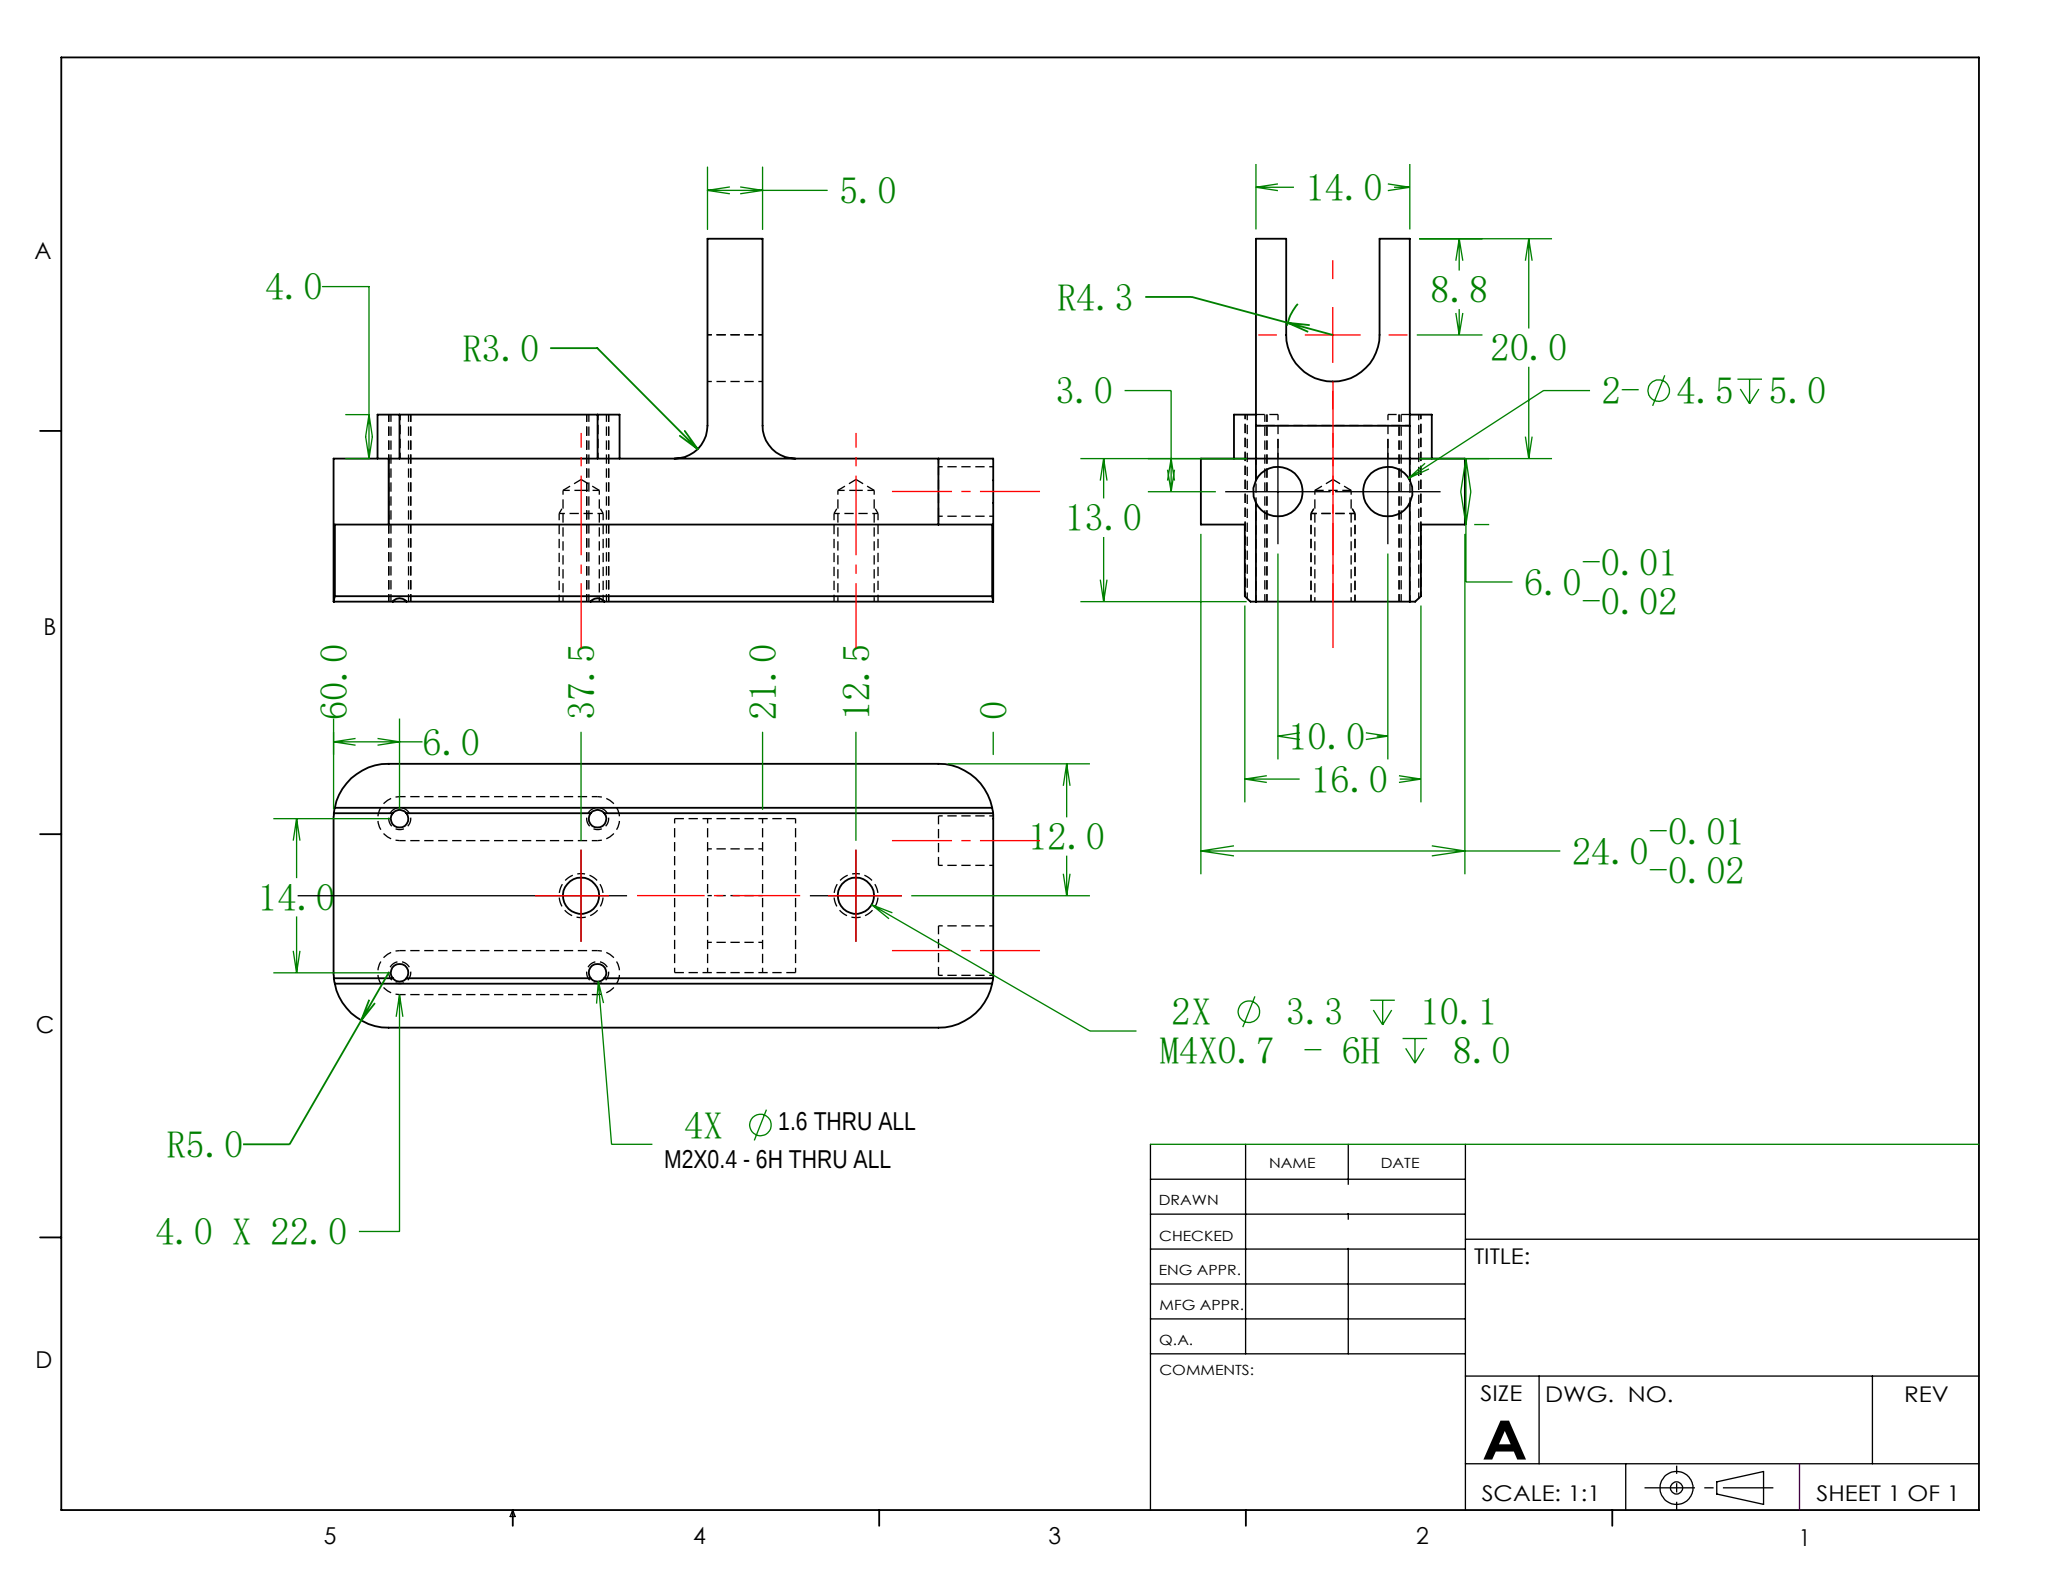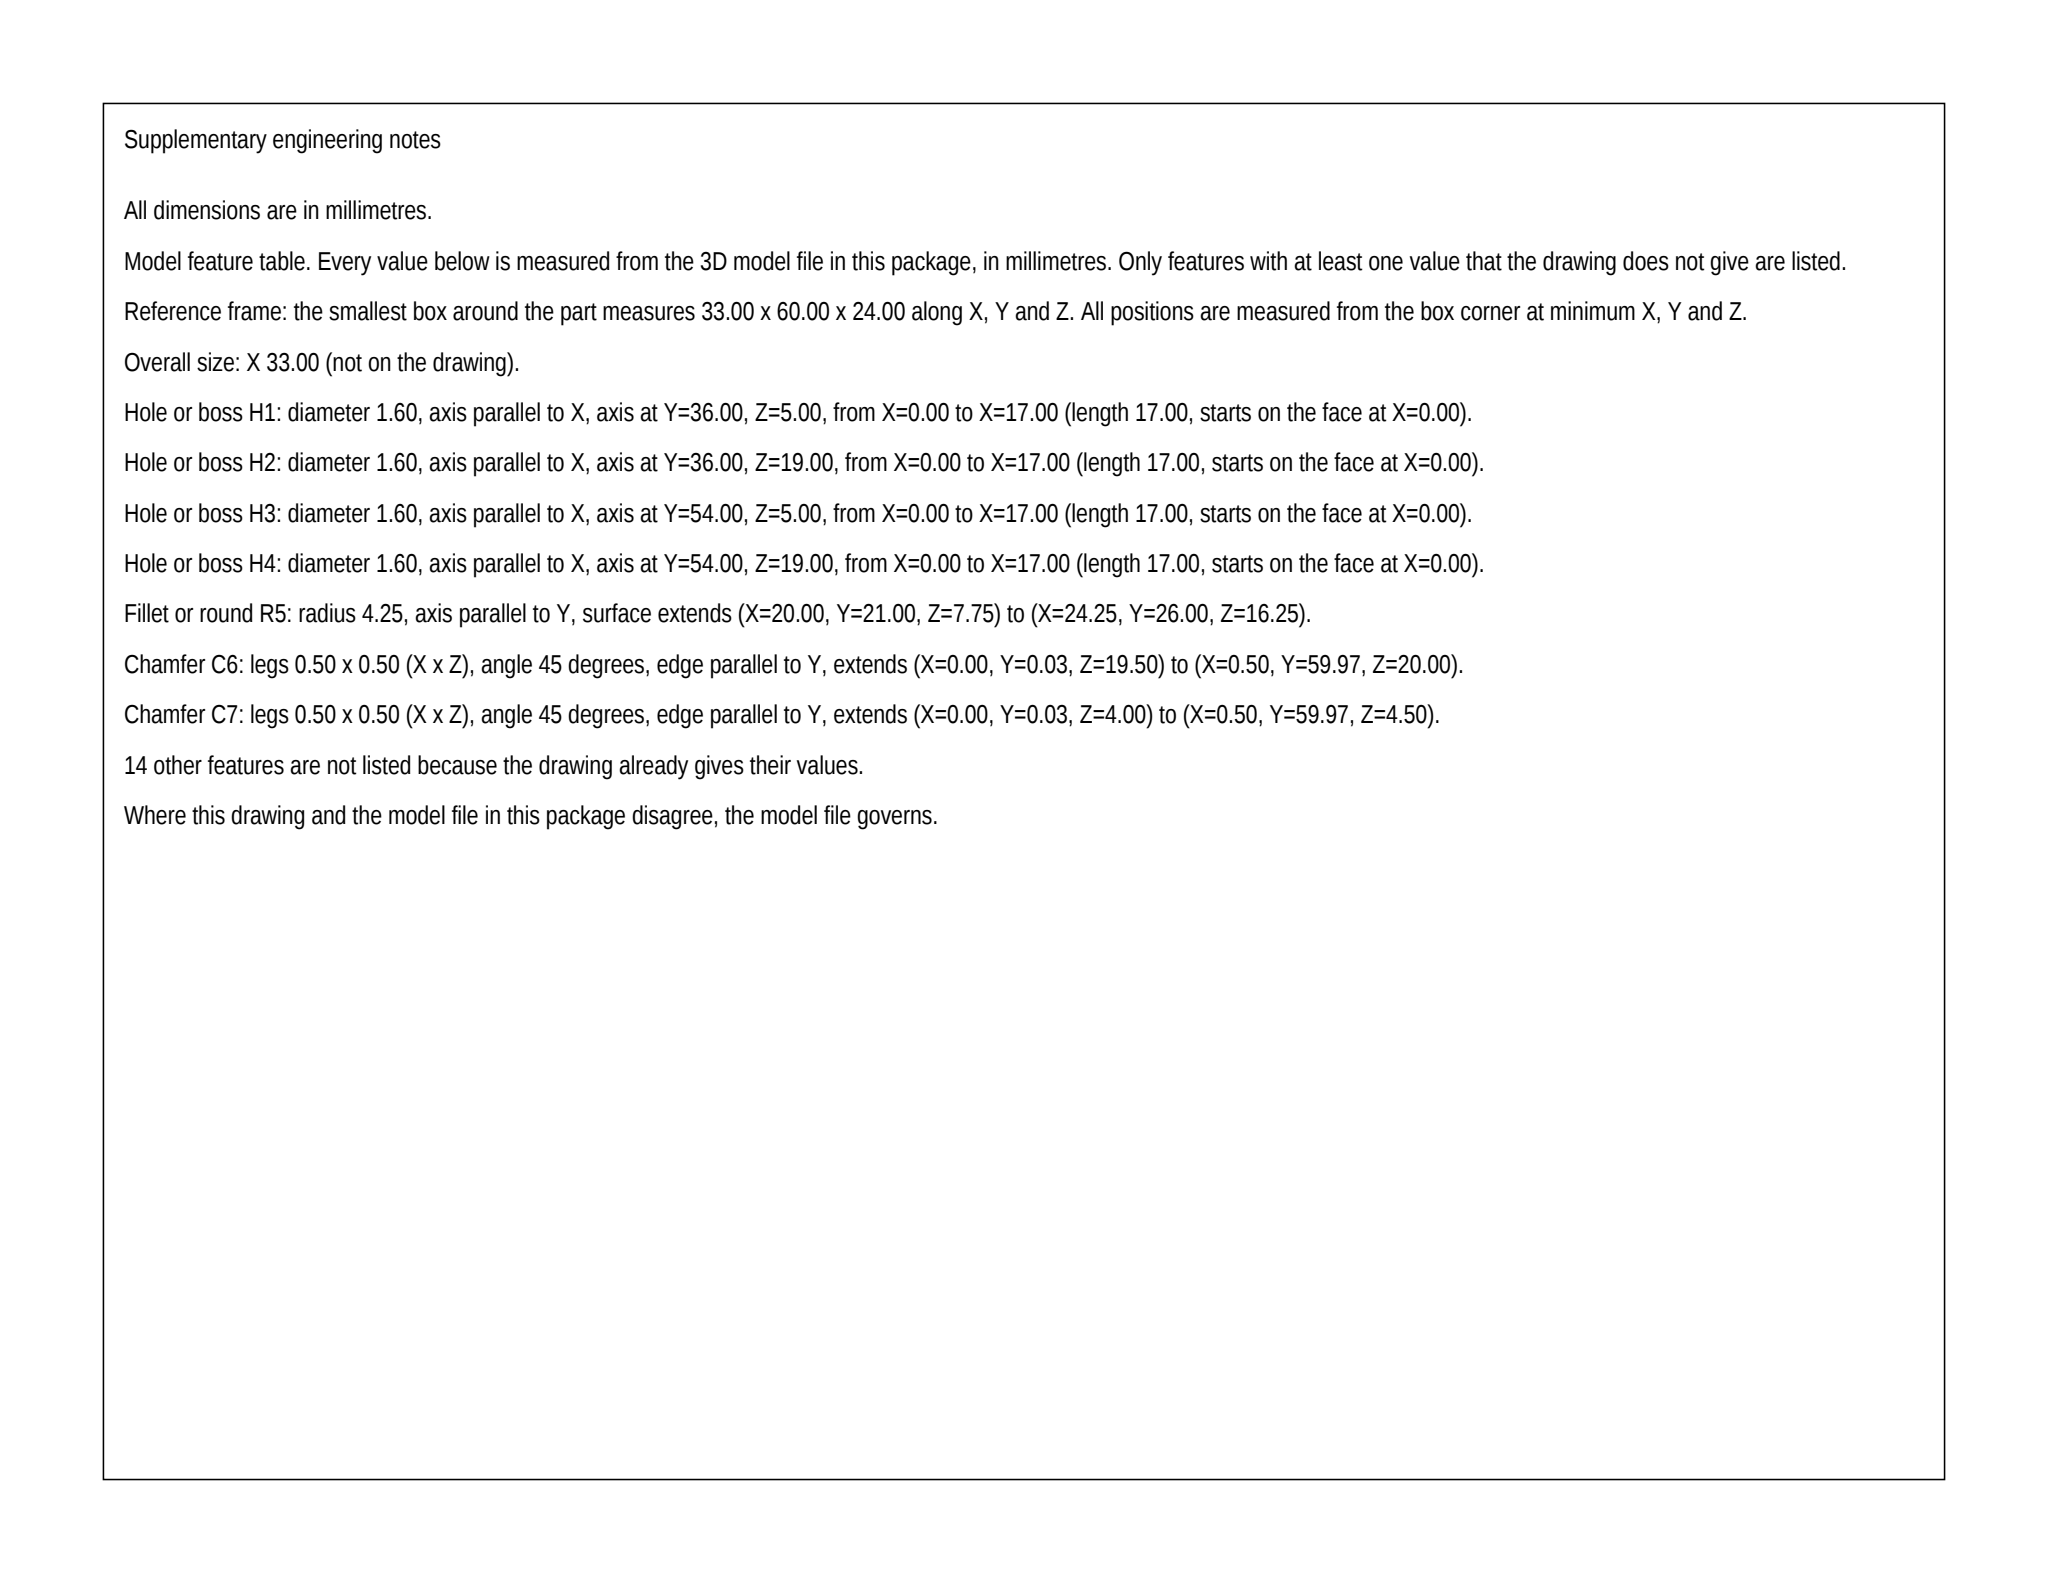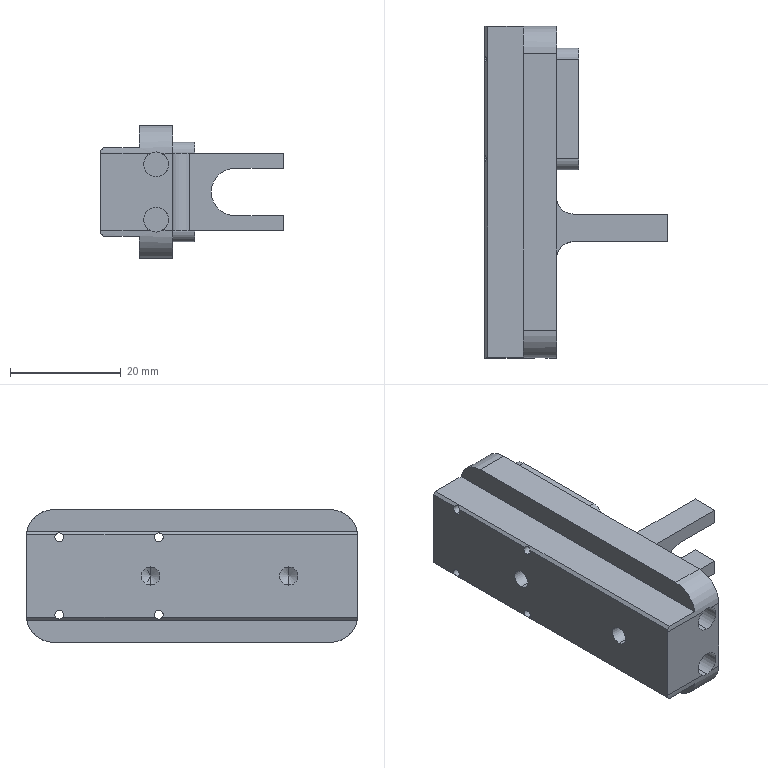Part | SolidWorks | mm | 1 solid | 60 faces | box 33 x 60 x 24 mm | volume 16358 mm3 | cylinder 28 | plane 28 | cone 4 | commonest cylinder face diameters 1.6 x8 3.3 x4 4.5 x4 4 x4 10 x4 8.5 x2 6 x2